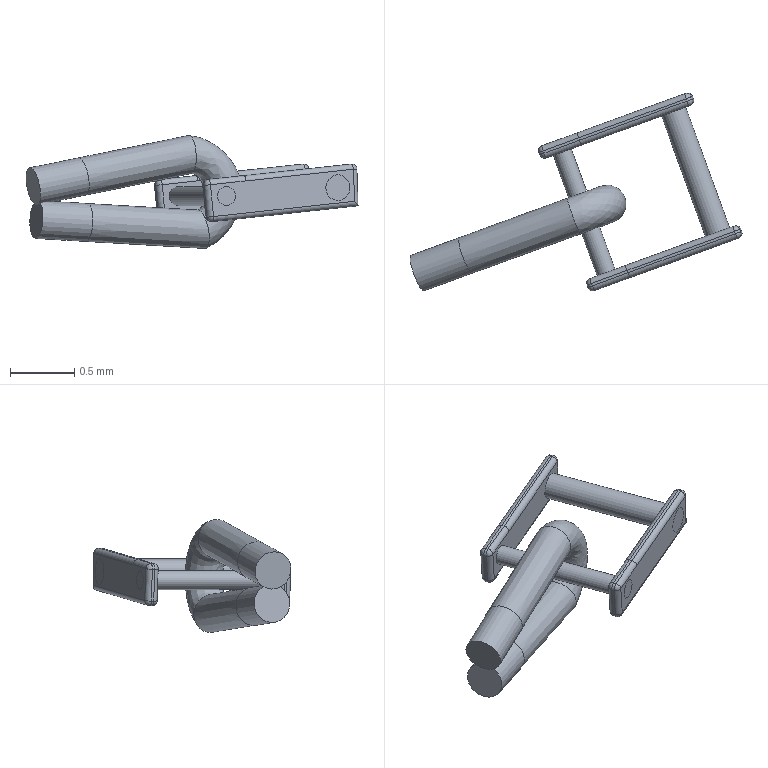Component | NX | MODEL11 | 5 solids | 70 faces | volume 0 mm3 | cylinder 35 | plane 20 | sphere 12 | spline 3 | commonest cylinder face diameters 0.08 x26 0.148 x4 0.2 x3 0.296 x2